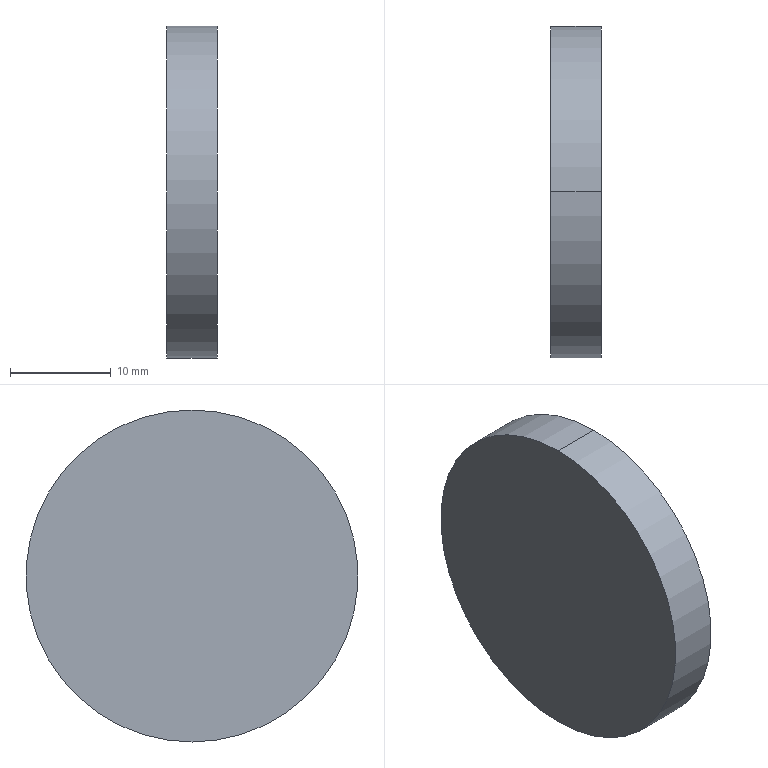Component | SolidWorks | JF21-110.1-34-1-SOLID1-1 | 1 solid | 4 faces | box 5 x 33 x 33 mm | volume 4276 mm3 | cylinder 2 | plane 2 | commonest cylinder face diameters 33 x2
STEP:
#1=COLOUR_RGB('',0.7922,0.8196,0.9333);
#2=FILL_AREA_STYLE_COLOUR('',#1);
#3=FILL_AREA_STYLE('',(#2));
#4=SURFACE_STYLE_FILL_AREA(#3);
#5=SURFACE_SIDE_STYLE('',(#4));
#6=SURFACE_STYLE_USAGE(.BOTH.,#5);
#7=PRESENTATION_STYLE_ASSIGNMENT((#6));
#8=CARTESIAN_POINT('',(17.252,-17.52,22.185));
#9=VERTEX_POINT('',#8);
#10=CARTESIAN_POINT('',(17.252,-17.52,23.484));
#11=VERTEX_POINT('',#10);
#12=CARTESIAN_POINT('',(17.252,-17.52,22.835));
#13=DIRECTION('',(1.,0.,0.));
#14=DIRECTION('',(0.,0.,-1.));
#15=AXIS2_PLACEMENT_3D('',#12,#13,#14);
#16=CIRCLE('',#15,0.6496);
#17=EDGE_CURVE('',#9,#11,#16,.T.);
#18=ORIENTED_EDGE('',*,*,#17,.F.);
#19=CARTESIAN_POINT('',(17.055,-17.52,22.185));
#20=VERTEX_POINT('',#19);
#21=CARTESIAN_POINT('',(17.252,-17.52,22.185));
#22=DIRECTION('',(-1.,0.,-0.));
#23=VECTOR('',#22,39.37);
#24=LINE('',#21,#23);
#25=EDGE_CURVE('',#9,#20,#24,.T.);
#26=ORIENTED_EDGE('',*,*,#25,.T.);
#27=CARTESIAN_POINT('',(17.055,-17.52,23.484));
#28=VERTEX_POINT('',#27);
#29=CARTESIAN_POINT('',(17.055,-17.52,22.835));
#30=DIRECTION('',(1.,0.,0.));
#31=DIRECTION('',(0.,0.,-1.));
#32=AXIS2_PLACEMENT_3D('',#29,#30,#31);
#33=CIRCLE('',#32,0.6496);
#34=EDGE_CURVE('',#20,#28,#33,.T.);
#35=ORIENTED_EDGE('',*,*,#34,.T.);
#36=CARTESIAN_POINT('',(17.252,-17.52,23.484));
#37=DIRECTION('',(-1.,0.,-0.));
#38=VECTOR('',#37,39.37);
#39=LINE('',#36,#38);
#40=EDGE_CURVE('',#11,#28,#39,.T.);
#41=ORIENTED_EDGE('',*,*,#40,.F.);
#42=EDGE_LOOP('',(#18,#26,#35,#41));
#43=FACE_OUTER_BOUND('',#42,.T.);
#44=CARTESIAN_POINT('',(17.252,-17.52,22.835));
#45=DIRECTION('',(-1.,0.,-0.));
#46=DIRECTION('',(0.,0.,-1.));
#47=AXIS2_PLACEMENT_3D('',#44,#45,#46);
#48=CYLINDRICAL_SURFACE('',#47,0.6496);
#49=ADVANCED_FACE('',(#43),#48,.T.);
#50=ORIENTED_EDGE('',*,*,#25,.F.);
#51=CARTESIAN_POINT('',(17.252,-17.52,22.835));
#52=DIRECTION('',(1.,0.,0.));
#53=DIRECTION('',(0.,0.,-1.));
#54=AXIS2_PLACEMENT_3D('',#51,#52,#53);
#55=CIRCLE('',#54,0.6496);
#56=EDGE_CURVE('',#11,#9,#55,.T.);
#57=ORIENTED_EDGE('',*,*,#56,.F.);
#58=ORIENTED_EDGE('',*,*,#40,.T.);
#59=CARTESIAN_POINT('',(17.055,-17.52,22.835));
#60=DIRECTION('',(1.,0.,0.));
#61=DIRECTION('',(0.,0.,-1.));
#62=AXIS2_PLACEMENT_3D('',#59,#60,#61);
#63=CIRCLE('',#62,0.6496);
#64=EDGE_CURVE('',#28,#20,#63,.T.);
#65=ORIENTED_EDGE('',*,*,#64,.T.);
#66=EDGE_LOOP('',(#50,#57,#58,#65));
#67=FACE_OUTER_BOUND('',#66,.T.);
#68=CARTESIAN_POINT('',(17.252,-17.52,22.835));
#69=DIRECTION('',(-1.,0.,-0.));
#70=DIRECTION('',(0.,0.,-1.));
#71=AXIS2_PLACEMENT_3D('',#68,#69,#70);
#72=CYLINDRICAL_SURFACE('',#71,0.6496);
#73=ADVANCED_FACE('',(#67),#72,.T.);
#74=ORIENTED_EDGE('',*,*,#56,.T.);
#75=ORIENTED_EDGE('',*,*,#17,.T.);
#76=EDGE_LOOP('',(#74,#75));
#77=FACE_OUTER_BOUND('',#76,.T.);
#78=CARTESIAN_POINT('',(17.252,-17.52,22.835));
#79=DIRECTION('',(1.,0.,0.));
#80=DIRECTION('',(-0.,0.,1.));
#81=AXIS2_PLACEMENT_3D('',#78,#79,#80);
#82=PLANE('',#81);
#83=ADVANCED_FACE('',(#77),#82,.T.);
#84=ORIENTED_EDGE('',*,*,#64,.F.);
#85=ORIENTED_EDGE('',*,*,#34,.F.);
#86=EDGE_LOOP('',(#84,#85));
#87=FACE_OUTER_BOUND('',#86,.T.);
#88=CARTESIAN_POINT('',(17.055,-17.52,22.835));
#89=DIRECTION('',(1.,0.,0.));
#90=DIRECTION('',(-0.,0.,1.));
#91=AXIS2_PLACEMENT_3D('',#88,#89,#90);
#92=PLANE('',#91);
#93=ADVANCED_FACE('',(#87),#92,.F.);
#94=CLOSED_SHELL('',(#49,#73,#83,#93));
#95=MANIFOLD_SOLID_BREP('',#94);
#96=STYLED_ITEM('',(#7),#95);
#97=(LENGTH_UNIT()NAMED_UNIT(*)SI_UNIT($,.METRE.));
#98=LENGTH_MEASURE_WITH_UNIT(LENGTH_MEASURE(0.0254),#97);
#99=DIMENSIONAL_EXPONENTS(1.,0.,0.,0.,0.,0.,0.);
#100=(CONVERSION_BASED_UNIT('',#98)LENGTH_UNIT()NAMED_UNIT(#99));
#101=UNCERTAINTY_MEASURE_WITH_UNIT(LENGTH_MEASURE(0.00001),#100,'','');
#102=(NAMED_UNIT(*)PLANE_ANGLE_UNIT()SI_UNIT($,.RADIAN.));
#103=(NAMED_UNIT(*)SI_UNIT($,.STERADIAN.)SOLID_ANGLE_UNIT());
#104=(GEOMETRIC_REPRESENTATION_CONTEXT(3)GLOBAL_UNCERTAINTY_ASSIGNED_CONTEXT((#101))GLOBAL_UNIT_ASSIGNED_CONTEXT((#100,#102,#103))REPRESENTATION_CONTEXT('',''));
#105=MECHANICAL_DESIGN_GEOMETRIC_PRESENTATION_REPRESENTATION('',(#96),#104);
#106=PRESENTATION_LAYER_ASSIGNMENT('','',(#96));
#107=CARTESIAN_POINT('',(0.,0.,0.));
#108=DIRECTION('',(0.,0.,1.));
#109=DIRECTION('',(1.,0.,0.));
#110=AXIS2_PLACEMENT_3D('',#107,#108,#109);
#111=(LENGTH_UNIT()NAMED_UNIT(*)SI_UNIT($,.METRE.));
#112=LENGTH_MEASURE_WITH_UNIT(LENGTH_MEASURE(0.0254),#111);
#113=DIMENSIONAL_EXPONENTS(1.,0.,0.,0.,0.,0.,0.);
#114=(CONVERSION_BASED_UNIT('',#112)LENGTH_UNIT()NAMED_UNIT(#113));
#115=UNCERTAINTY_MEASURE_WITH_UNIT(LENGTH_MEASURE(0.00001),#114,'','');
#116=(NAMED_UNIT(*)PLANE_ANGLE_UNIT()SI_UNIT($,.RADIAN.));
#117=(NAMED_UNIT(*)SI_UNIT($,.STERADIAN.)SOLID_ANGLE_UNIT());
#118=(GEOMETRIC_REPRESENTATION_CONTEXT(3)GLOBAL_UNCERTAINTY_ASSIGNED_CONTEXT((#115))GLOBAL_UNIT_ASSIGNED_CONTEXT((#114,#116,#117))REPRESENTATION_CONTEXT('',''));
#119=ADVANCED_BREP_SHAPE_REPRESENTATION('',(#95,#110),#118);